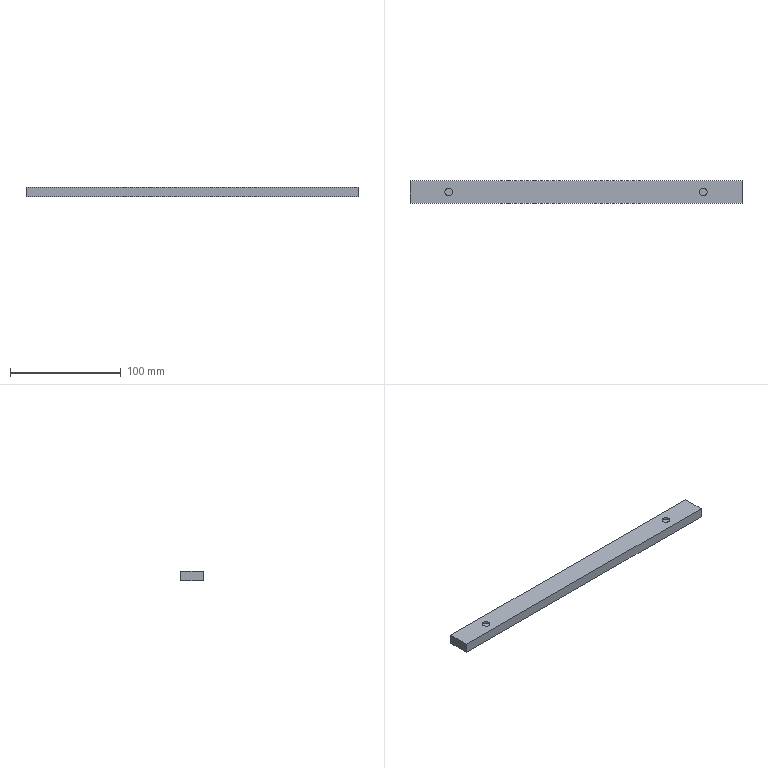Component | SolidWorks | 25ClampingGuidePlate-1 | 1 solid | 12 faces | box 300 x 20 x 9 mm | volume 53885 mm3 | plane 8 | cylinder 4 | commonest cylinder face diameters 7 x4
build123d program:
from build123d import *

# Parameters (mm, degrees)
SKETCH1_W           = 9
SKETCH1_H           = 20
BOSS_EXTRUDE1_DEPTH = 300
SKETCH2_R           = 3.5
CUT_EXTRUDE1_DEPTH  = 1.5


with BuildPart() as part:
    # Sketch1 → Boss-Extrude1 (new body)
    with BuildSketch(Plane.XY):
        Rectangle(SKETCH1_W, SKETCH1_H)
    extrude(amount=BOSS_EXTRUDE1_DEPTH)

    # Sketch2 → Cut-Extrude1 (cut)
    with BuildSketch(Plane(origin=(4.5, 0, 0), x_dir=(0, 0, -1), z_dir=(1, 0, 0))):
        with Locations(Location((-35, 0, 0), (0, 0, 90))):
            Circle(SKETCH2_R)
        with Locations(Location((-265, 0, 0), (0, 0, 90))):
            Circle(SKETCH2_R)
    extrude(amount=-CUT_EXTRUDE1_DEPTH, mode=Mode.SUBTRACT)


solid = part.part

# Placed as in the assembly
solid = solid.moved(Location((145.283, 145, -26.5), (0, -90, 0)))
STEP:
#1=CARTESIAN_POINT('',(-4.713,5.571,-0.9252));
#2=VERTEX_POINT('',#1);
#3=CARTESIAN_POINT('',(-4.713,5.846,-0.9252));
#4=VERTEX_POINT('',#3);
#5=CARTESIAN_POINT('',(-4.713,5.709,-0.9252));
#6=DIRECTION('',(0.,0.,1.));
#7=DIRECTION('',(0.,1.,0.));
#8=AXIS2_PLACEMENT_3D('',#5,#6,#7);
#9=CIRCLE('',#8,0.1378);
#10=EDGE_CURVE('',#2,#4,#9,.T.);
#11=ORIENTED_EDGE('',*,*,#10,.F.);
#12=CARTESIAN_POINT('',(-4.713,5.571,-0.8661));
#13=VERTEX_POINT('',#12);
#14=CARTESIAN_POINT('',(-4.713,5.571,-0.9252));
#15=DIRECTION('',(0.,0.,1.));
#16=VECTOR('',#15,39.37);
#17=LINE('',#14,#16);
#18=EDGE_CURVE('',#2,#13,#17,.T.);
#19=ORIENTED_EDGE('',*,*,#18,.T.);
#20=CARTESIAN_POINT('',(-4.713,5.846,-0.8661));
#21=VERTEX_POINT('',#20);
#22=CARTESIAN_POINT('',(-4.713,5.709,-0.8661));
#23=DIRECTION('',(0.,0.,1.));
#24=DIRECTION('',(0.,1.,0.));
#25=AXIS2_PLACEMENT_3D('',#22,#23,#24);
#26=CIRCLE('',#25,0.1378);
#27=EDGE_CURVE('',#13,#21,#26,.T.);
#28=ORIENTED_EDGE('',*,*,#27,.T.);
#29=CARTESIAN_POINT('',(-4.713,5.846,-0.9252));
#30=DIRECTION('',(0.,0.,1.));
#31=VECTOR('',#30,39.37);
#32=LINE('',#29,#31);
#33=EDGE_CURVE('',#4,#21,#32,.T.);
#34=ORIENTED_EDGE('',*,*,#33,.F.);
#35=EDGE_LOOP('',(#11,#19,#28,#34));
#36=FACE_OUTER_BOUND('',#35,.T.);
#37=CARTESIAN_POINT('',(-4.713,5.709,-0.9252));
#38=DIRECTION('',(0.,0.,1.));
#39=DIRECTION('',(0.,1.,0.));
#40=AXIS2_PLACEMENT_3D('',#37,#38,#39);
#41=CYLINDRICAL_SURFACE('',#40,0.1378);
#42=ADVANCED_FACE('',(#36),#41,.F.);
#43=CARTESIAN_POINT('',(4.342,5.571,-0.9252));
#44=VERTEX_POINT('',#43);
#45=CARTESIAN_POINT('',(4.342,5.846,-0.9252));
#46=VERTEX_POINT('',#45);
#47=CARTESIAN_POINT('',(4.342,5.709,-0.9252));
#48=DIRECTION('',(0.,0.,1.));
#49=DIRECTION('',(0.,1.,0.));
#50=AXIS2_PLACEMENT_3D('',#47,#48,#49);
#51=CIRCLE('',#50,0.1378);
#52=EDGE_CURVE('',#44,#46,#51,.T.);
#53=ORIENTED_EDGE('',*,*,#52,.F.);
#54=CARTESIAN_POINT('',(4.342,5.571,-0.8661));
#55=VERTEX_POINT('',#54);
#56=CARTESIAN_POINT('',(4.342,5.571,-0.9252));
#57=DIRECTION('',(0.,0.,1.));
#58=VECTOR('',#57,39.37);
#59=LINE('',#56,#58);
#60=EDGE_CURVE('',#44,#55,#59,.T.);
#61=ORIENTED_EDGE('',*,*,#60,.T.);
#62=CARTESIAN_POINT('',(4.342,5.846,-0.8661));
#63=VERTEX_POINT('',#62);
#64=CARTESIAN_POINT('',(4.342,5.709,-0.8661));
#65=DIRECTION('',(0.,0.,1.));
#66=DIRECTION('',(0.,1.,0.));
#67=AXIS2_PLACEMENT_3D('',#64,#65,#66);
#68=CIRCLE('',#67,0.1378);
#69=EDGE_CURVE('',#55,#63,#68,.T.);
#70=ORIENTED_EDGE('',*,*,#69,.T.);
#71=CARTESIAN_POINT('',(4.342,5.846,-0.9252));
#72=DIRECTION('',(0.,0.,1.));
#73=VECTOR('',#72,39.37);
#74=LINE('',#71,#73);
#75=EDGE_CURVE('',#46,#63,#74,.T.);
#76=ORIENTED_EDGE('',*,*,#75,.F.);
#77=EDGE_LOOP('',(#53,#61,#70,#76));
#78=FACE_OUTER_BOUND('',#77,.T.);
#79=CARTESIAN_POINT('',(4.342,5.709,-0.9252));
#80=DIRECTION('',(0.,0.,1.));
#81=DIRECTION('',(0.,1.,0.));
#82=AXIS2_PLACEMENT_3D('',#79,#80,#81);
#83=CYLINDRICAL_SURFACE('',#82,0.1378);
#84=ADVANCED_FACE('',(#78),#83,.F.);
#85=CARTESIAN_POINT('',(-4.713,5.709,-0.8661));
#86=DIRECTION('',(0.,0.,1.));
#87=DIRECTION('',(0.,1.,0.));
#88=AXIS2_PLACEMENT_3D('',#85,#86,#87);
#89=CIRCLE('',#88,0.1378);
#90=EDGE_CURVE('',#21,#13,#89,.T.);
#91=ORIENTED_EDGE('',*,*,#90,.F.);
#92=ORIENTED_EDGE('',*,*,#27,.F.);
#93=EDGE_LOOP('',(#91,#92));
#94=FACE_BOUND('',#93,.T.);
#95=CARTESIAN_POINT('',(4.342,5.709,-0.8661));
#96=DIRECTION('',(0.,0.,1.));
#97=DIRECTION('',(0.,1.,0.));
#98=AXIS2_PLACEMENT_3D('',#95,#96,#97);
#99=CIRCLE('',#98,0.1378);
#100=EDGE_CURVE('',#63,#55,#99,.T.);
#101=ORIENTED_EDGE('',*,*,#100,.F.);
#102=ORIENTED_EDGE('',*,*,#69,.F.);
#103=EDGE_LOOP('',(#101,#102));
#104=FACE_BOUND('',#103,.T.);
#105=CARTESIAN_POINT('',(5.72,5.315,-0.8661));
#106=VERTEX_POINT('',#105);
#107=CARTESIAN_POINT('',(5.72,6.102,-0.8661));
#108=VERTEX_POINT('',#107);
#109=CARTESIAN_POINT('',(5.72,6.102,-0.8661));
#110=DIRECTION('',(-0.,1.,-0.));
#111=VECTOR('',#110,39.37);
#112=LINE('',#109,#111);
#113=EDGE_CURVE('',#106,#108,#112,.T.);
#114=ORIENTED_EDGE('',*,*,#113,.T.);
#115=CARTESIAN_POINT('',(-6.091,6.102,-0.8661));
#116=VERTEX_POINT('',#115);
#117=CARTESIAN_POINT('',(-6.091,6.102,-0.8661));
#118=DIRECTION('',(1.,0.,-0.));
#119=VECTOR('',#118,39.37);
#120=LINE('',#117,#119);
#121=EDGE_CURVE('',#116,#108,#120,.T.);
#122=ORIENTED_EDGE('',*,*,#121,.F.);
#123=CARTESIAN_POINT('',(-6.091,5.315,-0.8661));
#124=VERTEX_POINT('',#123);
#125=CARTESIAN_POINT('',(-6.091,6.102,-0.8661));
#126=DIRECTION('',(-0.,1.,-0.));
#127=VECTOR('',#126,39.37);
#128=LINE('',#125,#127);
#129=EDGE_CURVE('',#124,#116,#128,.T.);
#130=ORIENTED_EDGE('',*,*,#129,.F.);
#131=CARTESIAN_POINT('',(-6.091,5.315,-0.8661));
#132=DIRECTION('',(1.,0.,-0.));
#133=VECTOR('',#132,39.37);
#134=LINE('',#131,#133);
#135=EDGE_CURVE('',#124,#106,#134,.T.);
#136=ORIENTED_EDGE('',*,*,#135,.T.);
#137=EDGE_LOOP('',(#114,#122,#130,#136));
#138=FACE_OUTER_BOUND('',#137,.T.);
#139=CARTESIAN_POINT('',(-6.091,6.102,-0.8661));
#140=DIRECTION('',(-0.,-0.,-1.));
#141=DIRECTION('',(0.,-1.,0.));
#142=AXIS2_PLACEMENT_3D('',#139,#140,#141);
#143=PLANE('',#142);
#144=ADVANCED_FACE('',(#94,#104,#138),#143,.F.);
#145=CARTESIAN_POINT('',(5.72,6.102,-1.22));
#146=VERTEX_POINT('',#145);
#147=CARTESIAN_POINT('',(5.72,6.102,-1.22));
#148=DIRECTION('',(-0.,-0.,-1.));
#149=VECTOR('',#148,39.37);
#150=LINE('',#147,#149);
#151=EDGE_CURVE('',#108,#146,#150,.T.);
#152=ORIENTED_EDGE('',*,*,#151,.T.);
#153=CARTESIAN_POINT('',(-6.091,6.102,-1.22));
#154=VERTEX_POINT('',#153);
#155=CARTESIAN_POINT('',(-6.091,6.102,-1.22));
#156=DIRECTION('',(1.,0.,-0.));
#157=VECTOR('',#156,39.37);
#158=LINE('',#155,#157);
#159=EDGE_CURVE('',#154,#146,#158,.T.);
#160=ORIENTED_EDGE('',*,*,#159,.F.);
#161=CARTESIAN_POINT('',(-6.091,6.102,-1.22));
#162=DIRECTION('',(-0.,-0.,-1.));
#163=VECTOR('',#162,39.37);
#164=LINE('',#161,#163);
#165=EDGE_CURVE('',#116,#154,#164,.T.);
#166=ORIENTED_EDGE('',*,*,#165,.F.);
#167=ORIENTED_EDGE('',*,*,#121,.T.);
#168=EDGE_LOOP('',(#152,#160,#166,#167));
#169=FACE_OUTER_BOUND('',#168,.T.);
#170=CARTESIAN_POINT('',(-6.091,6.102,-1.22));
#171=DIRECTION('',(0.,-1.,0.));
#172=DIRECTION('',(1.,0.,-0.));
#173=AXIS2_PLACEMENT_3D('',#170,#171,#172);
#174=PLANE('',#173);
#175=ADVANCED_FACE('',(#169),#174,.F.);
#176=CARTESIAN_POINT('',(5.72,5.315,-1.22));
#177=VERTEX_POINT('',#176);
#178=CARTESIAN_POINT('',(5.72,6.102,-1.22));
#179=DIRECTION('',(0.,-1.,0.));
#180=VECTOR('',#179,39.37);
#181=LINE('',#178,#180);
#182=EDGE_CURVE('',#146,#177,#181,.T.);
#183=ORIENTED_EDGE('',*,*,#182,.T.);
#184=CARTESIAN_POINT('',(-6.091,5.315,-1.22));
#185=VERTEX_POINT('',#184);
#186=CARTESIAN_POINT('',(-6.091,5.315,-1.22));
#187=DIRECTION('',(1.,0.,-0.));
#188=VECTOR('',#187,39.37);
#189=LINE('',#186,#188);
#190=EDGE_CURVE('',#185,#177,#189,.T.);
#191=ORIENTED_EDGE('',*,*,#190,.F.);
#192=CARTESIAN_POINT('',(-6.091,6.102,-1.22));
#193=DIRECTION('',(0.,-1.,0.));
#194=VECTOR('',#193,39.37);
#195=LINE('',#192,#194);
#196=EDGE_CURVE('',#154,#185,#195,.T.);
#197=ORIENTED_EDGE('',*,*,#196,.F.);
#198=ORIENTED_EDGE('',*,*,#159,.T.);
#199=EDGE_LOOP('',(#183,#191,#197,#198));
#200=FACE_OUTER_BOUND('',#199,.T.);
#201=CARTESIAN_POINT('',(-6.091,6.102,-1.22));
#202=DIRECTION('',(0.,0.,1.));
#203=DIRECTION('',(-0.,1.,-0.));
#204=AXIS2_PLACEMENT_3D('',#201,#202,#203);
#205=PLANE('',#204);
#206=ADVANCED_FACE('',(#200),#205,.F.);
#207=CARTESIAN_POINT('',(5.72,5.315,-1.22));
#208=DIRECTION('',(0.,0.,1.));
#209=VECTOR('',#208,39.37);
#210=LINE('',#207,#209);
#211=EDGE_CURVE('',#177,#106,#210,.T.);
#212=ORIENTED_EDGE('',*,*,#211,.T.);
#213=ORIENTED_EDGE('',*,*,#135,.F.);
#214=CARTESIAN_POINT('',(-6.091,5.315,-1.22));
#215=DIRECTION('',(0.,0.,1.));
#216=VECTOR('',#215,39.37);
#217=LINE('',#214,#216);
#218=EDGE_CURVE('',#185,#124,#217,.T.);
#219=ORIENTED_EDGE('',*,*,#218,.F.);
#220=ORIENTED_EDGE('',*,*,#190,.T.);
#221=EDGE_LOOP('',(#212,#213,#219,#220));
#222=FACE_OUTER_BOUND('',#221,.T.);
#223=CARTESIAN_POINT('',(-6.091,5.315,-1.22));
#224=DIRECTION('',(-0.,1.,-0.));
#225=DIRECTION('',(-1.,-0.,0.));
#226=AXIS2_PLACEMENT_3D('',#223,#224,#225);
#227=PLANE('',#226);
#228=ADVANCED_FACE('',(#222),#227,.F.);
#229=ORIENTED_EDGE('',*,*,#129,.T.);
#230=ORIENTED_EDGE('',*,*,#165,.T.);
#231=ORIENTED_EDGE('',*,*,#196,.T.);
#232=ORIENTED_EDGE('',*,*,#218,.T.);
#233=EDGE_LOOP('',(#229,#230,#231,#232));
#234=FACE_OUTER_BOUND('',#233,.T.);
#235=CARTESIAN_POINT('',(-6.091,5.709,-1.043));
#236=DIRECTION('',(-1.,-0.,0.));
#237=DIRECTION('',(0.,0.,1.));
#238=AXIS2_PLACEMENT_3D('',#235,#236,#237);
#239=PLANE('',#238);
#240=ADVANCED_FACE('',(#234),#239,.T.);
#241=ORIENTED_EDGE('',*,*,#113,.F.);
#242=ORIENTED_EDGE('',*,*,#211,.F.);
#243=ORIENTED_EDGE('',*,*,#182,.F.);
#244=ORIENTED_EDGE('',*,*,#151,.F.);
#245=EDGE_LOOP('',(#241,#242,#243,#244));
#246=FACE_OUTER_BOUND('',#245,.T.);
#247=CARTESIAN_POINT('',(5.72,5.709,-1.043));
#248=DIRECTION('',(-1.,-0.,0.));
#249=DIRECTION('',(0.,0.,1.));
#250=AXIS2_PLACEMENT_3D('',#247,#248,#249);
#251=PLANE('',#250);
#252=ADVANCED_FACE('',(#246),#251,.F.);
#253=ORIENTED_EDGE('',*,*,#60,.F.);
#254=CARTESIAN_POINT('',(4.342,5.709,-0.9252));
#255=DIRECTION('',(0.,0.,1.));
#256=DIRECTION('',(0.,1.,0.));
#257=AXIS2_PLACEMENT_3D('',#254,#255,#256);
#258=CIRCLE('',#257,0.1378);
#259=EDGE_CURVE('',#46,#44,#258,.T.);
#260=ORIENTED_EDGE('',*,*,#259,.F.);
#261=ORIENTED_EDGE('',*,*,#75,.T.);
#262=ORIENTED_EDGE('',*,*,#100,.T.);
#263=EDGE_LOOP('',(#253,#260,#261,#262));
#264=FACE_OUTER_BOUND('',#263,.T.);
#265=CARTESIAN_POINT('',(4.342,5.709,-0.9252));
#266=DIRECTION('',(0.,0.,1.));
#267=DIRECTION('',(0.,1.,0.));
#268=AXIS2_PLACEMENT_3D('',#265,#266,#267);
#269=CYLINDRICAL_SURFACE('',#268,0.1378);
#270=ADVANCED_FACE('',(#264),#269,.F.);
#271=ORIENTED_EDGE('',*,*,#259,.T.);
#272=ORIENTED_EDGE('',*,*,#52,.T.);
#273=EDGE_LOOP('',(#271,#272));
#274=FACE_OUTER_BOUND('',#273,.T.);
#275=CARTESIAN_POINT('',(4.342,5.709,-0.9252));
#276=DIRECTION('',(0.,0.,1.));
#277=DIRECTION('',(-0.,1.,-0.));
#278=AXIS2_PLACEMENT_3D('',#275,#276,#277);
#279=PLANE('',#278);
#280=ADVANCED_FACE('',(#274),#279,.T.);
#281=ORIENTED_EDGE('',*,*,#18,.F.);
#282=CARTESIAN_POINT('',(-4.713,5.709,-0.9252));
#283=DIRECTION('',(0.,0.,1.));
#284=DIRECTION('',(0.,1.,0.));
#285=AXIS2_PLACEMENT_3D('',#282,#283,#284);
#286=CIRCLE('',#285,0.1378);
#287=EDGE_CURVE('',#4,#2,#286,.T.);
#288=ORIENTED_EDGE('',*,*,#287,.F.);
#289=ORIENTED_EDGE('',*,*,#33,.T.);
#290=ORIENTED_EDGE('',*,*,#90,.T.);
#291=EDGE_LOOP('',(#281,#288,#289,#290));
#292=FACE_OUTER_BOUND('',#291,.T.);
#293=CARTESIAN_POINT('',(-4.713,5.709,-0.9252));
#294=DIRECTION('',(0.,0.,1.));
#295=DIRECTION('',(0.,1.,0.));
#296=AXIS2_PLACEMENT_3D('',#293,#294,#295);
#297=CYLINDRICAL_SURFACE('',#296,0.1378);
#298=ADVANCED_FACE('',(#292),#297,.F.);
#299=ORIENTED_EDGE('',*,*,#287,.T.);
#300=ORIENTED_EDGE('',*,*,#10,.T.);
#301=EDGE_LOOP('',(#299,#300));
#302=FACE_OUTER_BOUND('',#301,.T.);
#303=CARTESIAN_POINT('',(-4.713,5.709,-0.9252));
#304=DIRECTION('',(0.,0.,1.));
#305=DIRECTION('',(-0.,1.,-0.));
#306=AXIS2_PLACEMENT_3D('',#303,#304,#305);
#307=PLANE('',#306);
#308=ADVANCED_FACE('',(#302),#307,.T.);
#309=CLOSED_SHELL('',(#42,#84,#144,#175,#206,#228,#240,#252,#270,#280,#298,#308));
#310=MANIFOLD_SOLID_BREP('',#309);
#311=CARTESIAN_POINT('',(0.,0.,0.));
#312=DIRECTION('',(0.,0.,1.));
#313=DIRECTION('',(1.,0.,0.));
#314=AXIS2_PLACEMENT_3D('',#311,#312,#313);
#315=(LENGTH_UNIT()NAMED_UNIT(*)SI_UNIT($,.METRE.));
#316=LENGTH_MEASURE_WITH_UNIT(LENGTH_MEASURE(0.0254),#315);
#317=DIMENSIONAL_EXPONENTS(1.,0.,0.,0.,0.,0.,0.);
#318=(CONVERSION_BASED_UNIT('',#316)LENGTH_UNIT()NAMED_UNIT(#317));
#319=UNCERTAINTY_MEASURE_WITH_UNIT(LENGTH_MEASURE(0.00001),#318,'','');
#320=(NAMED_UNIT(*)PLANE_ANGLE_UNIT()SI_UNIT($,.RADIAN.));
#321=(NAMED_UNIT(*)SI_UNIT($,.STERADIAN.)SOLID_ANGLE_UNIT());
#322=(GEOMETRIC_REPRESENTATION_CONTEXT(3)GLOBAL_UNCERTAINTY_ASSIGNED_CONTEXT((#319))GLOBAL_UNIT_ASSIGNED_CONTEXT((#318,#320,#321))REPRESENTATION_CONTEXT('',''));
#323=ADVANCED_BREP_SHAPE_REPRESENTATION('',(#310,#314),#322);
#324=COLOUR_RGB('',0.7922,0.8196,0.9333);
#325=FILL_AREA_STYLE_COLOUR('',#324);
#326=FILL_AREA_STYLE('',(#325));
#327=SURFACE_STYLE_FILL_AREA(#326);
#328=SURFACE_SIDE_STYLE('',(#327));
#329=SURFACE_STYLE_USAGE(.BOTH.,#328);
#330=PRESENTATION_STYLE_ASSIGNMENT((#329));
#331=STYLED_ITEM('',(#330),#310);
#332=(LENGTH_UNIT()NAMED_UNIT(*)SI_UNIT($,.METRE.));
#333=LENGTH_MEASURE_WITH_UNIT(LENGTH_MEASURE(0.0254),#332);
#334=DIMENSIONAL_EXPONENTS(1.,0.,0.,0.,0.,0.,0.);
#335=(CONVERSION_BASED_UNIT('',#333)LENGTH_UNIT()NAMED_UNIT(#334));
#336=UNCERTAINTY_MEASURE_WITH_UNIT(LENGTH_MEASURE(0.00001),#335,'','');
#337=(NAMED_UNIT(*)PLANE_ANGLE_UNIT()SI_UNIT($,.RADIAN.));
#338=(NAMED_UNIT(*)SI_UNIT($,.STERADIAN.)SOLID_ANGLE_UNIT());
#339=(GEOMETRIC_REPRESENTATION_CONTEXT(3)GLOBAL_UNCERTAINTY_ASSIGNED_CONTEXT((#336))GLOBAL_UNIT_ASSIGNED_CONTEXT((#335,#337,#338))REPRESENTATION_CONTEXT('',''));
#340=MECHANICAL_DESIGN_GEOMETRIC_PRESENTATION_REPRESENTATION('',(#331),#339);
#341=PRESENTATION_LAYER_ASSIGNMENT('','',(#331));